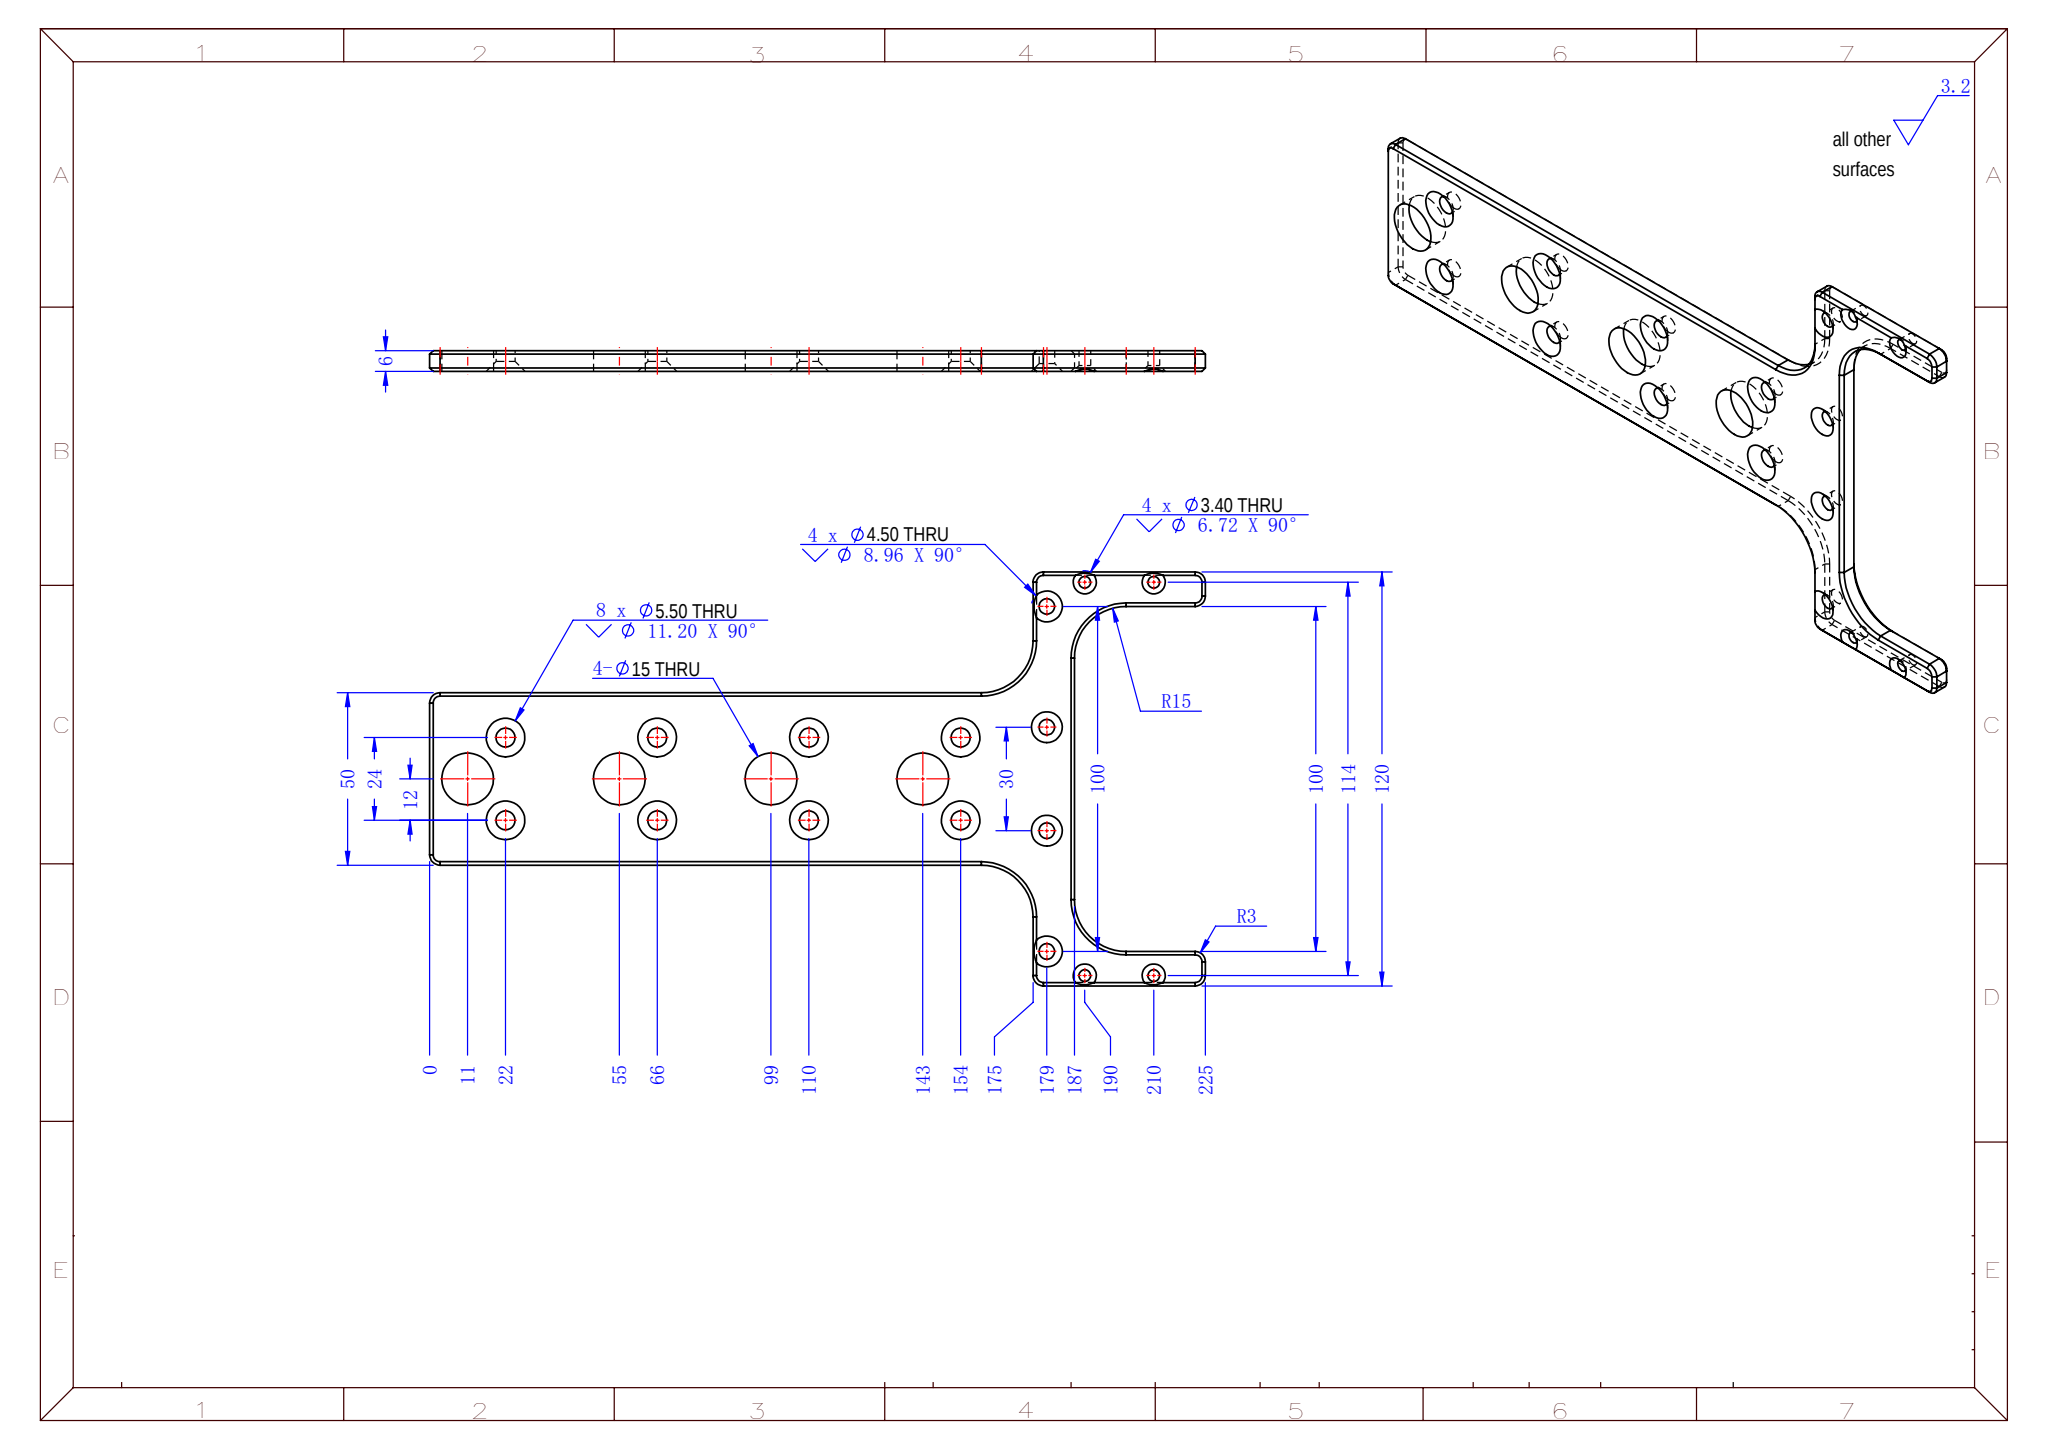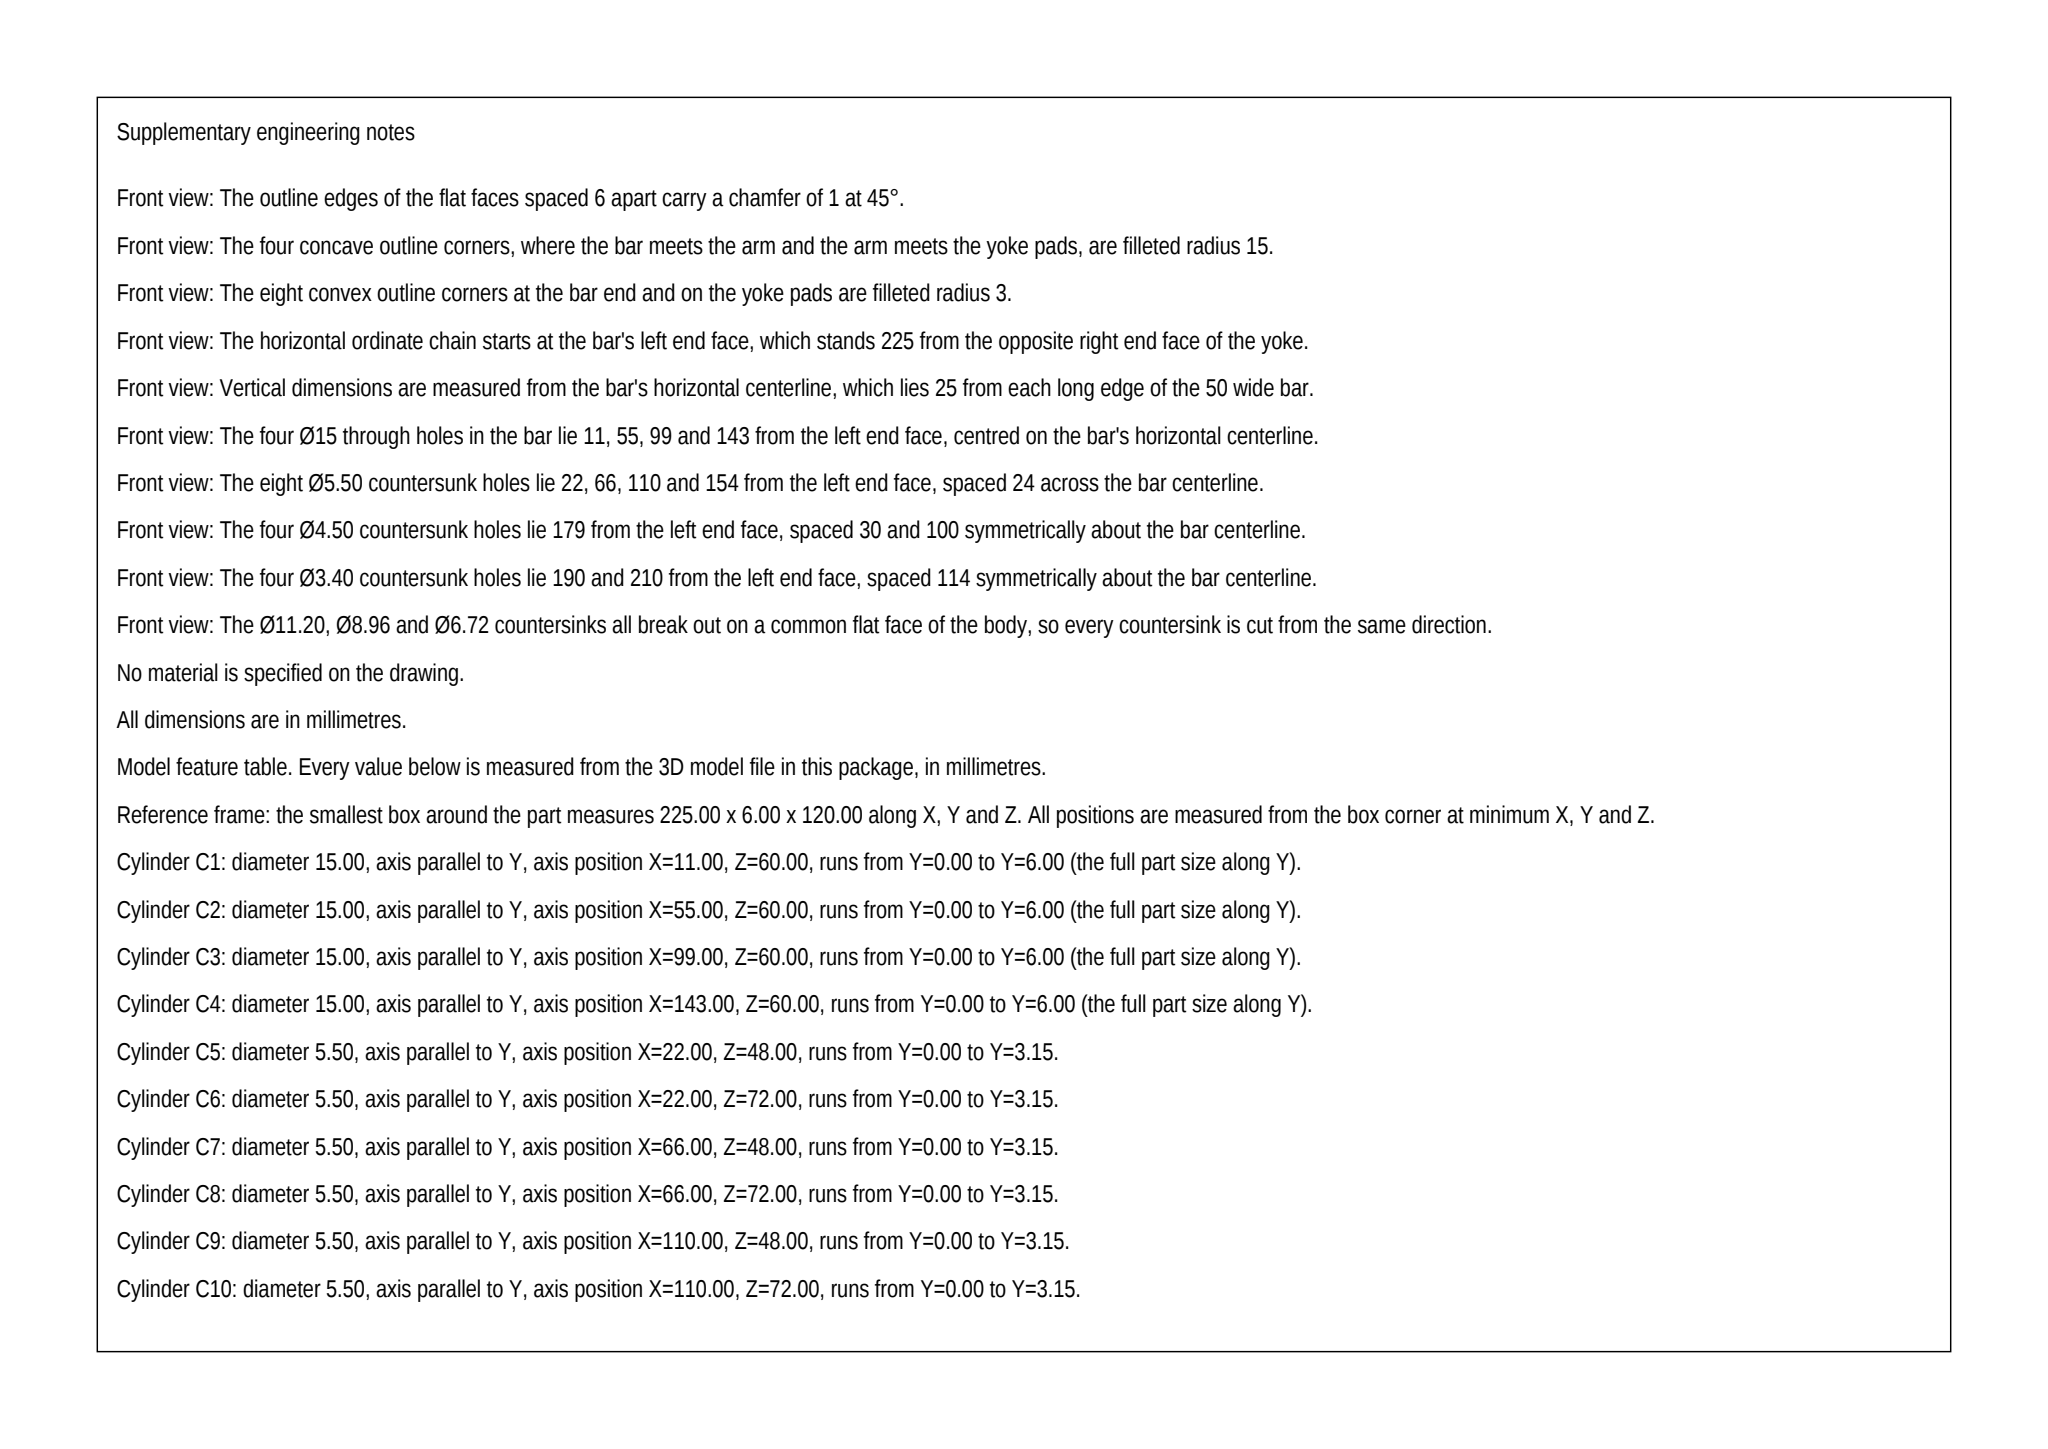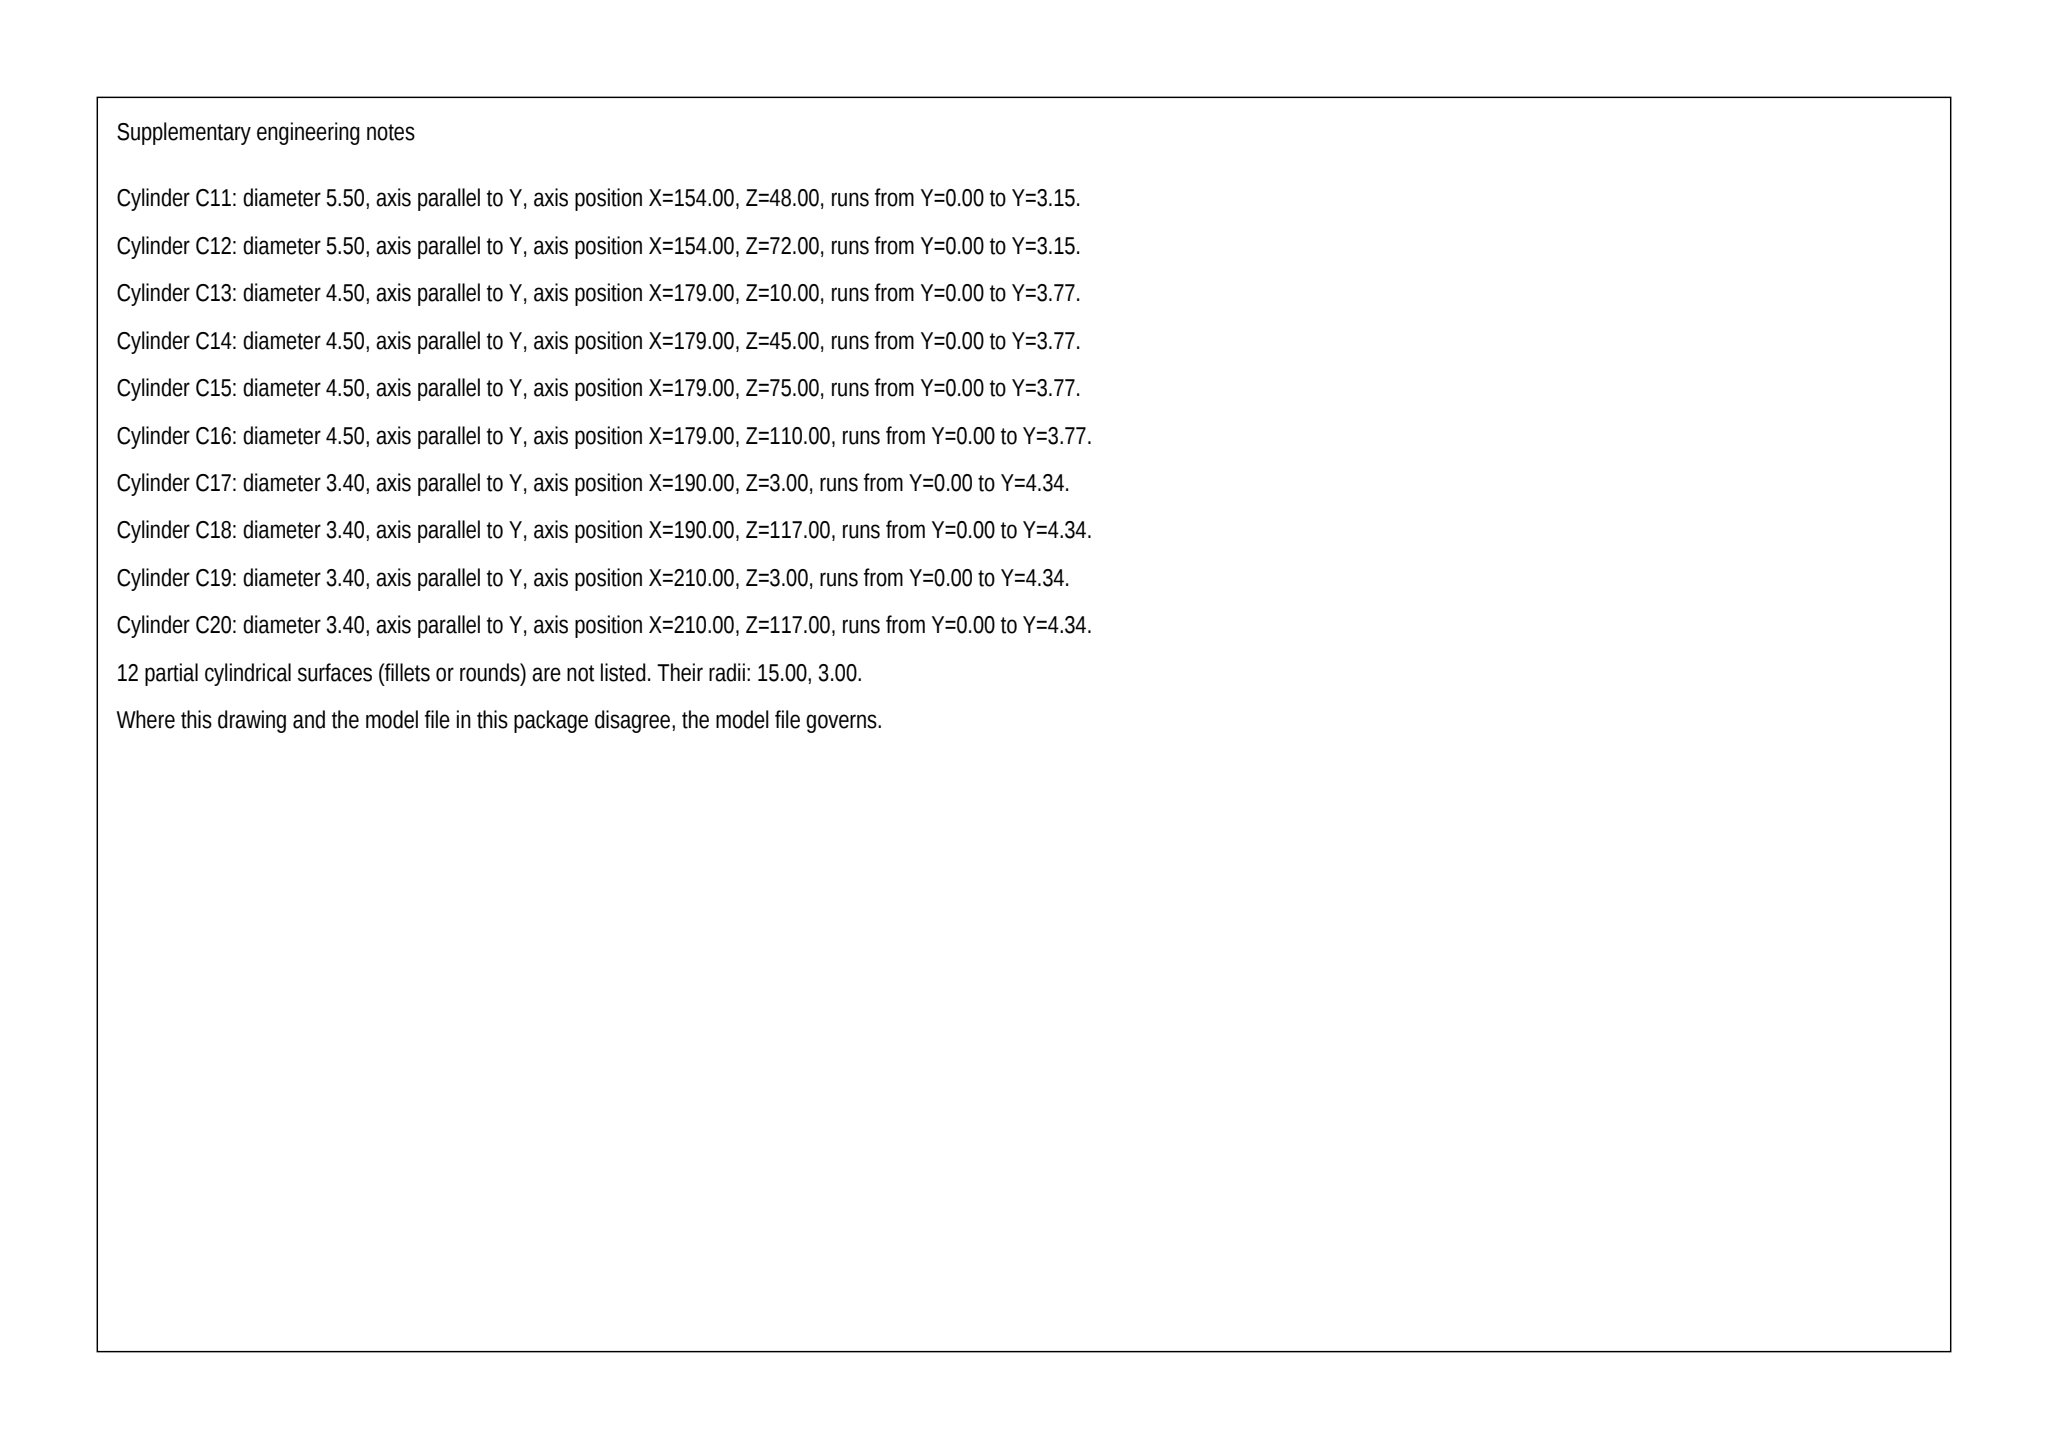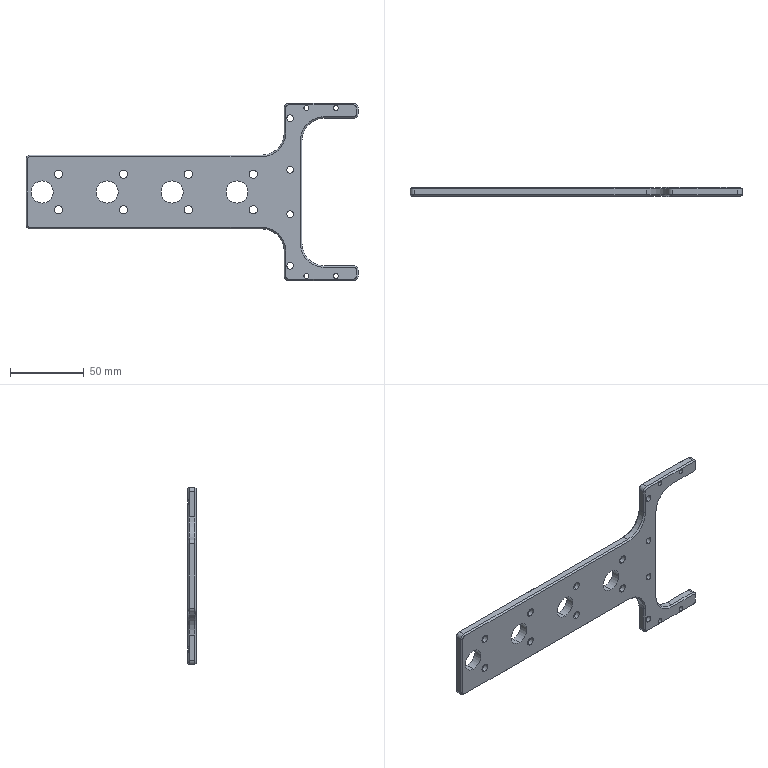Part | SolidWorks | mm | 1 solid | 146 faces | box 225 x 6 x 120 mm | volume 59046 mm3 | cone 56 | cylinder 52 | plane 38 | commonest cylinder face diameters 5.5 x16 3.4 x8 4.5 x8 15 x8 6 x8 30 x4
Drawing notes:
1 X 45° CHAMFER ALL AROUND PLATE OUTLINE, BOTH FACES | from the solid: 24 inclined planes at 45°/45°, 1.0 x 1.0 section, on y=0 and y=5 (6 thk) along full outline incl. R3 & R15 corners
R3 TYP 8 PLCS; R15 TYP 4 PLCS | from the solid: 8 convex arcs dia 6.0 (R3) at x3/178/222; 4 concave arcs dia 30.0 (R15) at (160,100.4),(160,20.4),(202,25.4),(202,95.4)